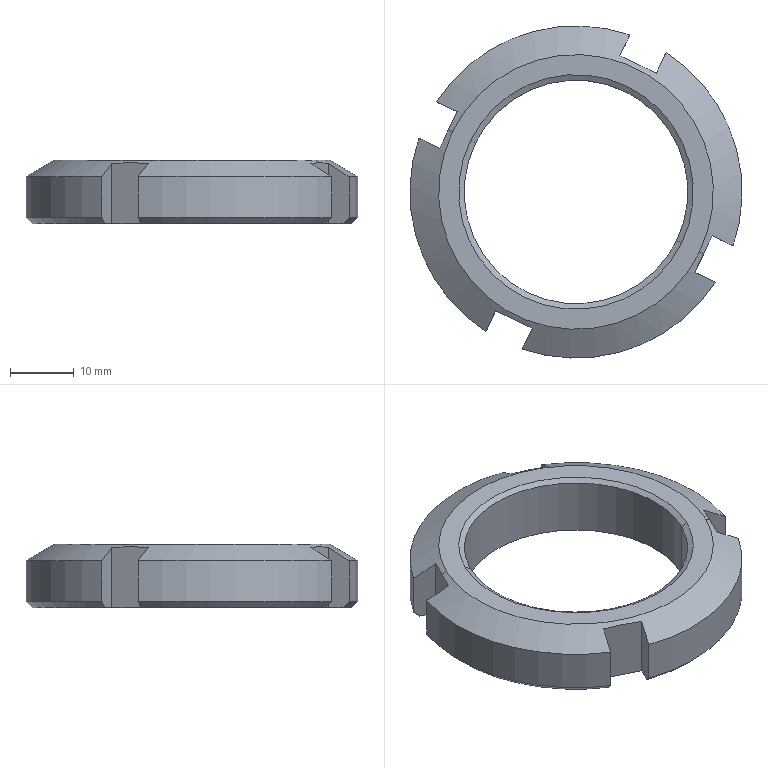Component | SolidWorks | GB812RoundNutM35_1.5-1 | 1 solid | 30 faces | box 52 x 52 x 10 mm | volume 9804 mm3 | plane 14 | cone 10 | cylinder 6 | commonest cylinder face diameters 52 x4 35 x2 | material A3
STEP:
#1=COLOUR_RGB('',0.7922,0.8196,0.9333);
#2=FILL_AREA_STYLE_COLOUR('',#1);
#3=FILL_AREA_STYLE('',(#2));
#4=SURFACE_STYLE_FILL_AREA(#3);
#5=SURFACE_SIDE_STYLE('',(#4));
#6=SURFACE_STYLE_USAGE(.BOTH.,#5);
#7=PRESENTATION_STYLE_ASSIGNMENT((#6));
#8=CARTESIAN_POINT('',(28.24,8.203,-0.07874));
#9=VERTEX_POINT('',#8);
#10=CARTESIAN_POINT('',(29.479,7.602,-0.07874));
#11=VERTEX_POINT('',#10);
#12=CARTESIAN_POINT('',(28.859,7.902,-0.07874));
#13=DIRECTION('',(0.,-0.,-1.));
#14=DIRECTION('',(0.8996,-0.4367,0.));
#15=AXIS2_PLACEMENT_3D('',#12,#13,#14);
#16=CIRCLE('',#15,0.689);
#17=EDGE_CURVE('',#9,#11,#16,.T.);
#18=ORIENTED_EDGE('',*,*,#17,.F.);
#19=CARTESIAN_POINT('',(28.209,8.218,-0.09843));
#20=VERTEX_POINT('',#19);
#21=CARTESIAN_POINT('',(28.24,8.203,-0.07874));
#22=DIRECTION('',(-0.7791,0.3782,-0.5));
#23=VECTOR('',#22,39.37);
#24=LINE('',#21,#23);
#25=EDGE_CURVE('',#9,#20,#24,.T.);
#26=ORIENTED_EDGE('',*,*,#25,.T.);
#27=CARTESIAN_POINT('',(29.51,7.587,-0.09843));
#28=VERTEX_POINT('',#27);
#29=CARTESIAN_POINT('',(28.859,7.902,-0.09843));
#30=DIRECTION('',(-0.,0.,1.));
#31=DIRECTION('',(0.8996,-0.4367,0.));
#32=AXIS2_PLACEMENT_3D('',#29,#30,#31);
#33=CIRCLE('',#32,0.7231);
#34=EDGE_CURVE('',#28,#20,#33,.T.);
#35=ORIENTED_EDGE('',*,*,#34,.F.);
#36=CARTESIAN_POINT('',(29.479,7.602,-0.07874));
#37=DIRECTION('',(0.7791,-0.3782,-0.5));
#38=VECTOR('',#37,39.37);
#39=LINE('',#36,#38);
#40=EDGE_CURVE('',#11,#28,#39,.T.);
#41=ORIENTED_EDGE('',*,*,#40,.F.);
#42=EDGE_LOOP('',(#18,#26,#35,#41));
#43=FACE_OUTER_BOUND('',#42,.T.);
#44=CARTESIAN_POINT('',(28.859,7.902,-0.07874));
#45=DIRECTION('',(0.,-0.,-1.));
#46=DIRECTION('',(0.8996,-0.4367,0.));
#47=AXIS2_PLACEMENT_3D('',#44,#45,#46);
#48=CONICAL_SURFACE('',#47,0.689,1.047);
#49=ADVANCED_FACE('',(#43),#48,.F.);
#50=CARTESIAN_POINT('',(29.479,7.602,0.2756));
#51=VERTEX_POINT('',#50);
#52=CARTESIAN_POINT('',(28.24,8.203,0.2756));
#53=VERTEX_POINT('',#52);
#54=CARTESIAN_POINT('',(28.859,7.902,0.2756));
#55=DIRECTION('',(-0.,0.,1.));
#56=DIRECTION('',(0.8996,-0.4367,0.));
#57=AXIS2_PLACEMENT_3D('',#54,#55,#56);
#58=CIRCLE('',#57,0.689);
#59=EDGE_CURVE('',#51,#53,#58,.T.);
#60=ORIENTED_EDGE('',*,*,#59,.F.);
#61=CARTESIAN_POINT('',(29.51,7.587,0.2953));
#62=VERTEX_POINT('',#61);
#63=CARTESIAN_POINT('',(29.51,7.587,0.2953));
#64=DIRECTION('',(0.7791,-0.3782,0.5));
#65=VECTOR('',#64,39.37);
#66=LINE('',#63,#65);
#67=EDGE_CURVE('',#51,#62,#66,.T.);
#68=ORIENTED_EDGE('',*,*,#67,.T.);
#69=CARTESIAN_POINT('',(28.209,8.218,0.2953));
#70=VERTEX_POINT('',#69);
#71=CARTESIAN_POINT('',(28.859,7.902,0.2953));
#72=DIRECTION('',(0.,-0.,-1.));
#73=DIRECTION('',(0.8996,-0.4367,0.));
#74=AXIS2_PLACEMENT_3D('',#71,#72,#73);
#75=CIRCLE('',#74,0.7231);
#76=EDGE_CURVE('',#70,#62,#75,.T.);
#77=ORIENTED_EDGE('',*,*,#76,.F.);
#78=CARTESIAN_POINT('',(28.209,8.218,0.2953));
#79=DIRECTION('',(-0.7791,0.3782,0.5));
#80=VECTOR('',#79,39.37);
#81=LINE('',#78,#80);
#82=EDGE_CURVE('',#53,#70,#81,.T.);
#83=ORIENTED_EDGE('',*,*,#82,.F.);
#84=EDGE_LOOP('',(#60,#68,#77,#83));
#85=FACE_OUTER_BOUND('',#84,.T.);
#86=CARTESIAN_POINT('',(28.859,7.902,0.2953));
#87=DIRECTION('',(-0.,0.,1.));
#88=DIRECTION('',(-0.8996,0.4367,-0.));
#89=AXIS2_PLACEMENT_3D('',#86,#87,#88);
#90=CONICAL_SURFACE('',#89,0.7231,1.047);
#91=ADVANCED_FACE('',(#85),#90,.F.);
#92=CARTESIAN_POINT('',(28.098,8.272,0.2953));
#93=VERTEX_POINT('',#92);
#94=CARTESIAN_POINT('',(29.621,7.533,0.2953));
#95=VERTEX_POINT('',#94);
#96=CARTESIAN_POINT('',(28.859,7.902,0.2953));
#97=DIRECTION('',(-0.,0.,1.));
#98=DIRECTION('',(0.8996,-0.4367,0.));
#99=AXIS2_PLACEMENT_3D('',#96,#97,#98);
#100=CIRCLE('',#99,0.8465);
#101=EDGE_CURVE('',#93,#95,#100,.T.);
#102=ORIENTED_EDGE('',*,*,#101,.F.);
#103=CARTESIAN_POINT('',(28.073,8.284,0.2792));
#104=VERTEX_POINT('',#103);
#105=CARTESIAN_POINT('',(27.939,8.349,0.193));
#106=DIRECTION('',(-0.7791,0.3782,-0.5));
#107=VECTOR('',#106,39.37);
#108=LINE('',#105,#107);
#109=EDGE_CURVE('',#93,#104,#108,.T.);
#110=ORIENTED_EDGE('',*,*,#109,.T.);
#111=CARTESIAN_POINT('',(28.019,8.173,0.2741));
#112=VERTEX_POINT('',#111);
#113=CARTESIAN_POINT('',(28.019,8.173,0.2741));
#114=CARTESIAN_POINT('',(28.037,8.21,0.2775));
#115=CARTESIAN_POINT('',(28.055,8.247,0.2792));
#116=CARTESIAN_POINT('',(28.073,8.284,0.2792));
#117=B_SPLINE_CURVE_WITH_KNOTS('',3,(#113,#114,#115,#116),.UNSPECIFIED.,.F.,.F.,(4,4),(0.006603,0.009752),.UNSPECIFIED.);
#118=EDGE_CURVE('',#112,#104,#117,.T.);
#119=ORIENTED_EDGE('',*,*,#118,.F.);
#120=CARTESIAN_POINT('',(27.891,8.235,0.193));
#121=VERTEX_POINT('',#120);
#122=CARTESIAN_POINT('',(27.891,8.235,0.193));
#123=CARTESIAN_POINT('',(27.934,8.214,0.2201));
#124=CARTESIAN_POINT('',(27.976,8.193,0.2471));
#125=CARTESIAN_POINT('',(28.019,8.173,0.2741));
#126=B_SPLINE_CURVE_WITH_KNOTS('',3,(#122,#123,#124,#125),.UNSPECIFIED.,.F.,.F.,(4,4),(0.007772,0.01192),.UNSPECIFIED.);
#127=EDGE_CURVE('',#121,#112,#126,.T.);
#128=ORIENTED_EDGE('',*,*,#127,.F.);
#129=CARTESIAN_POINT('',(28.304,7.043,0.193));
#130=VERTEX_POINT('',#129);
#131=CARTESIAN_POINT('',(28.859,7.902,0.193));
#132=DIRECTION('',(0.,-0.,-1.));
#133=DIRECTION('',(0.8996,-0.4367,0.));
#134=AXIS2_PLACEMENT_3D('',#131,#132,#133);
#135=CIRCLE('',#134,1.024);
#136=EDGE_CURVE('',#130,#121,#135,.T.);
#137=ORIENTED_EDGE('',*,*,#136,.F.);
#138=CARTESIAN_POINT('',(28.366,7.17,0.2741));
#139=VERTEX_POINT('',#138);
#140=CARTESIAN_POINT('',(28.366,7.17,0.2741));
#141=CARTESIAN_POINT('',(28.345,7.128,0.2471));
#142=CARTESIAN_POINT('',(28.325,7.085,0.2201));
#143=CARTESIAN_POINT('',(28.304,7.043,0.193));
#144=B_SPLINE_CURVE_WITH_KNOTS('',3,(#140,#141,#142,#143),.UNSPECIFIED.,.F.,.F.,(4,4),(0.008039,0.01219),.UNSPECIFIED.);
#145=EDGE_CURVE('',#139,#130,#144,.T.);
#146=ORIENTED_EDGE('',*,*,#145,.F.);
#147=CARTESIAN_POINT('',(28.589,7.062,0.2741));
#148=VERTEX_POINT('',#147);
#149=CARTESIAN_POINT('',(28.589,7.062,0.2741));
#150=CARTESIAN_POINT('',(28.552,7.08,0.2774));
#151=CARTESIAN_POINT('',(28.515,7.098,0.2792));
#152=CARTESIAN_POINT('',(28.459,7.125,0.2792));
#153=CARTESIAN_POINT('',(28.441,7.134,0.2788));
#154=CARTESIAN_POINT('',(28.403,7.152,0.2771));
#155=CARTESIAN_POINT('',(28.385,7.161,0.2758));
#156=CARTESIAN_POINT('',(28.366,7.17,0.2741));
#157=B_SPLINE_CURVE_WITH_KNOTS('',3,(#149,#150,#151,#152,#153,#154,#155,#156),.UNSPECIFIED.,.F.,.F.,(4,2,2,4),(0.006603,0.009741,0.01131,0.01288),.UNSPECIFIED.);
#158=EDGE_CURVE('',#148,#139,#157,.T.);
#159=ORIENTED_EDGE('',*,*,#158,.F.);
#160=CARTESIAN_POINT('',(28.527,6.934,0.193));
#161=VERTEX_POINT('',#160);
#162=CARTESIAN_POINT('',(28.527,6.934,0.193));
#163=CARTESIAN_POINT('',(28.548,6.977,0.2201));
#164=CARTESIAN_POINT('',(28.568,7.019,0.2471));
#165=CARTESIAN_POINT('',(28.589,7.062,0.2741));
#166=B_SPLINE_CURVE_WITH_KNOTS('',3,(#162,#163,#164,#165),.UNSPECIFIED.,.F.,.F.,(4,4),(0.004784,0.008932),.UNSPECIFIED.);
#167=EDGE_CURVE('',#161,#148,#166,.T.);
#168=ORIENTED_EDGE('',*,*,#167,.F.);
#169=CARTESIAN_POINT('',(29.719,7.347,0.193));
#170=VERTEX_POINT('',#169);
#171=CARTESIAN_POINT('',(28.859,7.902,0.193));
#172=DIRECTION('',(0.,-0.,-1.));
#173=DIRECTION('',(0.8996,-0.4367,0.));
#174=AXIS2_PLACEMENT_3D('',#171,#172,#173);
#175=CIRCLE('',#174,1.024);
#176=EDGE_CURVE('',#170,#161,#175,.T.);
#177=ORIENTED_EDGE('',*,*,#176,.F.);
#178=CARTESIAN_POINT('',(29.592,7.409,0.2741));
#179=VERTEX_POINT('',#178);
#180=CARTESIAN_POINT('',(29.592,7.409,0.2741));
#181=CARTESIAN_POINT('',(29.634,7.388,0.2471));
#182=CARTESIAN_POINT('',(29.677,7.368,0.2201));
#183=CARTESIAN_POINT('',(29.719,7.347,0.193));
#184=B_SPLINE_CURVE_WITH_KNOTS('',3,(#180,#181,#182,#183),.UNSPECIFIED.,.F.,.F.,(4,4),(0.008039,0.01219),.UNSPECIFIED.);
#185=EDGE_CURVE('',#179,#170,#184,.T.);
#186=ORIENTED_EDGE('',*,*,#185,.F.);
#187=CARTESIAN_POINT('',(29.646,7.521,0.2792));
#188=VERTEX_POINT('',#187);
#189=CARTESIAN_POINT('',(29.646,7.521,0.2792));
#190=CARTESIAN_POINT('',(29.628,7.483,0.2792));
#191=CARTESIAN_POINT('',(29.61,7.446,0.2775));
#192=CARTESIAN_POINT('',(29.592,7.409,0.2741));
#193=B_SPLINE_CURVE_WITH_KNOTS('',3,(#189,#190,#191,#192),.UNSPECIFIED.,.F.,.F.,(4,4),(0.01618,0.01933),.UNSPECIFIED.);
#194=EDGE_CURVE('',#188,#179,#193,.T.);
#195=ORIENTED_EDGE('',*,*,#194,.F.);
#196=CARTESIAN_POINT('',(29.78,7.455,0.193));
#197=DIRECTION('',(0.7791,-0.3782,-0.5));
#198=VECTOR('',#197,39.37);
#199=LINE('',#196,#198);
#200=EDGE_CURVE('',#95,#188,#199,.T.);
#201=ORIENTED_EDGE('',*,*,#200,.F.);
#202=EDGE_LOOP('',(#102,#110,#119,#128,#137,#146,#159,#168,#177,#186,#195,#201));
#203=FACE_OUTER_BOUND('',#202,.T.);
#204=CARTESIAN_POINT('',(28.859,7.902,0.193));
#205=DIRECTION('',(0.,-0.,-1.));
#206=DIRECTION('',(0.8996,-0.4367,0.));
#207=AXIS2_PLACEMENT_3D('',#204,#205,#206);
#208=CONICAL_SURFACE('',#207,1.024,1.047);
#209=ADVANCED_FACE('',(#203),#208,.T.);
#210=ORIENTED_EDGE('',*,*,#17,.T.);
#211=CARTESIAN_POINT('',(29.479,7.602,-0.09843));
#212=DIRECTION('',(-0.,0.,1.));
#213=VECTOR('',#212,39.37);
#214=LINE('',#211,#213);
#215=EDGE_CURVE('',#11,#51,#214,.T.);
#216=ORIENTED_EDGE('',*,*,#215,.T.);
#217=ORIENTED_EDGE('',*,*,#59,.T.);
#218=CARTESIAN_POINT('',(28.24,8.203,-0.09843));
#219=DIRECTION('',(-0.,0.,1.));
#220=VECTOR('',#219,39.37);
#221=LINE('',#218,#220);
#222=EDGE_CURVE('',#9,#53,#221,.T.);
#223=ORIENTED_EDGE('',*,*,#222,.F.);
#224=EDGE_LOOP('',(#210,#216,#217,#223));
#225=FACE_OUTER_BOUND('',#224,.T.);
#226=CARTESIAN_POINT('',(28.859,7.902,-0.09843));
#227=DIRECTION('',(-0.,0.,1.));
#228=DIRECTION('',(-0.8996,0.4367,-0.));
#229=AXIS2_PLACEMENT_3D('',#226,#227,#228);
#230=CYLINDRICAL_SURFACE('',#229,0.689);
#231=ADVANCED_FACE('',(#225),#230,.F.);
#232=CARTESIAN_POINT('',(28.527,6.934,-0.05906));
#233=VERTEX_POINT('',#232);
#234=CARTESIAN_POINT('',(29.719,7.347,-0.05906));
#235=VERTEX_POINT('',#234);
#236=CARTESIAN_POINT('',(28.859,7.902,-0.05906));
#237=DIRECTION('',(-0.,0.,1.));
#238=DIRECTION('',(0.8996,-0.4367,0.));
#239=AXIS2_PLACEMENT_3D('',#236,#237,#238);
#240=CIRCLE('',#239,1.024);
#241=EDGE_CURVE('',#233,#235,#240,.T.);
#242=ORIENTED_EDGE('',*,*,#241,.T.);
#243=CARTESIAN_POINT('',(29.719,7.347,0.2953));
#244=DIRECTION('',(0.,-0.,-1.));
#245=VECTOR('',#244,39.37);
#246=LINE('',#243,#245);
#247=EDGE_CURVE('',#170,#235,#246,.T.);
#248=ORIENTED_EDGE('',*,*,#247,.F.);
#249=ORIENTED_EDGE('',*,*,#176,.T.);
#250=CARTESIAN_POINT('',(28.527,6.934,0.2953));
#251=DIRECTION('',(0.,-0.,-1.));
#252=VECTOR('',#251,39.37);
#253=LINE('',#250,#252);
#254=EDGE_CURVE('',#161,#233,#253,.T.);
#255=ORIENTED_EDGE('',*,*,#254,.T.);
#256=EDGE_LOOP('',(#242,#248,#249,#255));
#257=FACE_OUTER_BOUND('',#256,.T.);
#258=CARTESIAN_POINT('',(28.859,7.902,-0.09843));
#259=DIRECTION('',(-0.,0.,1.));
#260=DIRECTION('',(-0.8996,0.4367,-0.));
#261=AXIS2_PLACEMENT_3D('',#258,#259,#260);
#262=CYLINDRICAL_SURFACE('',#261,1.024);
#263=ADVANCED_FACE('',(#257),#262,.T.);
#264=CARTESIAN_POINT('',(29.684,7.364,-0.09843));
#265=VERTEX_POINT('',#264);
#266=CARTESIAN_POINT('',(29.719,7.347,-0.05906));
#267=CARTESIAN_POINT('',(29.708,7.352,-0.07117));
#268=CARTESIAN_POINT('',(29.697,7.358,-0.08329));
#269=CARTESIAN_POINT('',(29.686,7.363,-0.0954));
#270=CARTESIAN_POINT('',(29.685,7.364,-0.09641));
#271=CARTESIAN_POINT('',(29.685,7.364,-0.09742));
#272=CARTESIAN_POINT('',(29.684,7.364,-0.09843));
#273=B_SPLINE_CURVE_WITH_KNOTS('',3,(#266,#267,#268,#269,#270,#271,#272),.UNSPECIFIED.,.F.,.F.,(4,3,4),(0.00583,0.007141,0.00725),.UNSPECIFIED.);
#274=EDGE_CURVE('',#235,#265,#273,.T.);
#275=ORIENTED_EDGE('',*,*,#274,.F.);
#276=ORIENTED_EDGE('',*,*,#241,.F.);
#277=CARTESIAN_POINT('',(28.545,6.97,-0.09843));
#278=VERTEX_POINT('',#277);
#279=CARTESIAN_POINT('',(28.545,6.97,-0.09843));
#280=CARTESIAN_POINT('',(28.544,6.969,-0.09742));
#281=CARTESIAN_POINT('',(28.544,6.968,-0.09641));
#282=CARTESIAN_POINT('',(28.543,6.967,-0.0954));
#283=CARTESIAN_POINT('',(28.538,6.956,-0.08329));
#284=CARTESIAN_POINT('',(28.533,6.945,-0.07117));
#285=CARTESIAN_POINT('',(28.527,6.934,-0.05906));
#286=B_SPLINE_CURVE_WITH_KNOTS('',3,(#279,#280,#281,#282,#283,#284,#285),.UNSPECIFIED.,.F.,.F.,(4,3,4),(0.007032,0.007141,0.008451),.UNSPECIFIED.);
#287=EDGE_CURVE('',#278,#233,#286,.T.);
#288=ORIENTED_EDGE('',*,*,#287,.F.);
#289=CARTESIAN_POINT('',(28.859,7.902,-0.09843));
#290=DIRECTION('',(0.,-0.,-1.));
#291=DIRECTION('',(0.8996,-0.4367,0.));
#292=AXIS2_PLACEMENT_3D('',#289,#290,#291);
#293=CIRCLE('',#292,0.9843);
#294=EDGE_CURVE('',#265,#278,#293,.T.);
#295=ORIENTED_EDGE('',*,*,#294,.F.);
#296=EDGE_LOOP('',(#275,#276,#288,#295));
#297=FACE_OUTER_BOUND('',#296,.T.);
#298=CARTESIAN_POINT('',(28.859,7.902,-0.09843));
#299=DIRECTION('',(-0.,0.,1.));
#300=DIRECTION('',(-0.8996,0.4367,-0.));
#301=AXIS2_PLACEMENT_3D('',#298,#299,#300);
#302=CONICAL_SURFACE('',#301,0.9843,0.7854);
#303=ADVANCED_FACE('',(#297),#302,.T.);
#304=CARTESIAN_POINT('',(27.891,8.235,-0.05906));
#305=VERTEX_POINT('',#304);
#306=CARTESIAN_POINT('',(28.304,7.043,-0.05906));
#307=VERTEX_POINT('',#306);
#308=CARTESIAN_POINT('',(28.859,7.902,-0.05906));
#309=DIRECTION('',(-0.,0.,1.));
#310=DIRECTION('',(0.8996,-0.4367,0.));
#311=AXIS2_PLACEMENT_3D('',#308,#309,#310);
#312=CIRCLE('',#311,1.024);
#313=EDGE_CURVE('',#305,#307,#312,.T.);
#314=ORIENTED_EDGE('',*,*,#313,.T.);
#315=CARTESIAN_POINT('',(28.304,7.043,0.2953));
#316=DIRECTION('',(0.,-0.,-1.));
#317=VECTOR('',#316,39.37);
#318=LINE('',#315,#317);
#319=EDGE_CURVE('',#130,#307,#318,.T.);
#320=ORIENTED_EDGE('',*,*,#319,.F.);
#321=ORIENTED_EDGE('',*,*,#136,.T.);
#322=CARTESIAN_POINT('',(27.891,8.235,0.2953));
#323=DIRECTION('',(0.,-0.,-1.));
#324=VECTOR('',#323,39.37);
#325=LINE('',#322,#324);
#326=EDGE_CURVE('',#121,#305,#325,.T.);
#327=ORIENTED_EDGE('',*,*,#326,.T.);
#328=EDGE_LOOP('',(#314,#320,#321,#327));
#329=FACE_OUTER_BOUND('',#328,.T.);
#330=CARTESIAN_POINT('',(28.859,7.902,-0.09843));
#331=DIRECTION('',(-0.,0.,1.));
#332=DIRECTION('',(-0.8996,0.4367,-0.));
#333=AXIS2_PLACEMENT_3D('',#330,#331,#332);
#334=CYLINDRICAL_SURFACE('',#333,1.024);
#335=ADVANCED_FACE('',(#329),#334,.T.);
#336=CARTESIAN_POINT('',(28.321,7.078,-0.09843));
#337=VERTEX_POINT('',#336);
#338=CARTESIAN_POINT('',(28.304,7.043,-0.05906));
#339=CARTESIAN_POINT('',(28.309,7.054,-0.07117));
#340=CARTESIAN_POINT('',(28.315,7.065,-0.08329));
#341=CARTESIAN_POINT('',(28.32,7.075,-0.0954));
#342=CARTESIAN_POINT('',(28.321,7.076,-0.09641));
#343=CARTESIAN_POINT('',(28.321,7.077,-0.09742));
#344=CARTESIAN_POINT('',(28.321,7.078,-0.09843));
#345=B_SPLINE_CURVE_WITH_KNOTS('',3,(#338,#339,#340,#341,#342,#343,#344),.UNSPECIFIED.,.F.,.F.,(4,3,4),(0.00583,0.007141,0.00725),.UNSPECIFIED.);
#346=EDGE_CURVE('',#307,#337,#345,.T.);
#347=ORIENTED_EDGE('',*,*,#346,.F.);
#348=ORIENTED_EDGE('',*,*,#313,.F.);
#349=CARTESIAN_POINT('',(27.927,8.217,-0.09843));
#350=VERTEX_POINT('',#349);
#351=CARTESIAN_POINT('',(27.927,8.217,-0.09843));
#352=CARTESIAN_POINT('',(27.921,8.22,-0.09151));
#353=CARTESIAN_POINT('',(27.914,8.223,-0.0846));
#354=CARTESIAN_POINT('',(27.908,8.226,-0.07768));
#355=CARTESIAN_POINT('',(27.902,8.229,-0.07147));
#356=CARTESIAN_POINT('',(27.897,8.232,-0.06526));
#357=CARTESIAN_POINT('',(27.891,8.235,-0.05906));
#358=B_SPLINE_CURVE_WITH_KNOTS('',3,(#351,#352,#353,#354,#355,#356,#357),.UNSPECIFIED.,.F.,.F.,(4,3,4),(0.006393,0.007141,0.007812),.UNSPECIFIED.);
#359=EDGE_CURVE('',#350,#305,#358,.T.);
#360=ORIENTED_EDGE('',*,*,#359,.F.);
#361=CARTESIAN_POINT('',(28.859,7.902,-0.09843));
#362=DIRECTION('',(0.,-0.,-1.));
#363=DIRECTION('',(0.8996,-0.4367,0.));
#364=AXIS2_PLACEMENT_3D('',#361,#362,#363);
#365=CIRCLE('',#364,0.9843);
#366=EDGE_CURVE('',#337,#350,#365,.T.);
#367=ORIENTED_EDGE('',*,*,#366,.F.);
#368=EDGE_LOOP('',(#347,#348,#360,#367));
#369=FACE_OUTER_BOUND('',#368,.T.);
#370=CARTESIAN_POINT('',(28.859,7.902,-0.09843));
#371=DIRECTION('',(-0.,0.,1.));
#372=DIRECTION('',(-0.8996,0.4367,-0.));
#373=AXIS2_PLACEMENT_3D('',#370,#371,#372);
#374=CONICAL_SURFACE('',#373,0.9843,0.7854);
#375=ADVANCED_FACE('',(#369),#374,.T.);
#376=CARTESIAN_POINT('',(29.192,8.871,-0.05906));
#377=VERTEX_POINT('',#376);
#378=CARTESIAN_POINT('',(28.,8.458,-0.05906));
#379=VERTEX_POINT('',#378);
#380=CARTESIAN_POINT('',(28.859,7.902,-0.05906));
#381=DIRECTION('',(-0.,0.,1.));
#382=DIRECTION('',(0.8996,-0.4367,0.));
#383=AXIS2_PLACEMENT_3D('',#380,#381,#382);
#384=CIRCLE('',#383,1.024);
#385=EDGE_CURVE('',#377,#379,#384,.T.);
#386=ORIENTED_EDGE('',*,*,#385,.T.);
#387=CARTESIAN_POINT('',(28.,8.458,0.193));
#388=VERTEX_POINT('',#387);
#389=CARTESIAN_POINT('',(28.,8.458,0.2953));
#390=DIRECTION('',(0.,-0.,-1.));
#391=VECTOR('',#390,39.37);
#392=LINE('',#389,#391);
#393=EDGE_CURVE('',#388,#379,#392,.T.);
#394=ORIENTED_EDGE('',*,*,#393,.F.);
#395=CARTESIAN_POINT('',(29.192,8.871,0.193));
#396=VERTEX_POINT('',#395);
#397=CARTESIAN_POINT('',(28.859,7.902,0.193));
#398=DIRECTION('',(0.,-0.,-1.));
#399=DIRECTION('',(0.8996,-0.4367,0.));
#400=AXIS2_PLACEMENT_3D('',#397,#398,#399);
#401=CIRCLE('',#400,1.024);
#402=EDGE_CURVE('',#388,#396,#401,.T.);
#403=ORIENTED_EDGE('',*,*,#402,.T.);
#404=CARTESIAN_POINT('',(29.192,8.871,0.2953));
#405=DIRECTION('',(0.,-0.,-1.));
#406=VECTOR('',#405,39.37);
#407=LINE('',#404,#406);
#408=EDGE_CURVE('',#396,#377,#407,.T.);
#409=ORIENTED_EDGE('',*,*,#408,.T.);
#410=EDGE_LOOP('',(#386,#394,#403,#409));
#411=FACE_OUTER_BOUND('',#410,.T.);
#412=CARTESIAN_POINT('',(28.859,7.902,-0.09843));
#413=DIRECTION('',(-0.,0.,1.));
#414=DIRECTION('',(-0.8996,0.4367,-0.));
#415=AXIS2_PLACEMENT_3D('',#412,#413,#414);
#416=CYLINDRICAL_SURFACE('',#415,1.024);
#417=ADVANCED_FACE('',(#411),#416,.T.);
#418=CARTESIAN_POINT('',(28.035,8.44,-0.09843));
#419=VERTEX_POINT('',#418);
#420=CARTESIAN_POINT('',(28.,8.458,-0.05906));
#421=CARTESIAN_POINT('',(28.005,8.455,-0.06526));
#422=CARTESIAN_POINT('',(28.011,8.452,-0.07147));
#423=CARTESIAN_POINT('',(28.016,8.45,-0.07768));
#424=CARTESIAN_POINT('',(28.023,8.447,-0.0846));
#425=CARTESIAN_POINT('',(28.029,8.443,-0.09151));
#426=CARTESIAN_POINT('',(28.035,8.44,-0.09843));
#427=B_SPLINE_CURVE_WITH_KNOTS('',3,(#420,#421,#422,#423,#424,#425,#426),.UNSPECIFIED.,.F.,.F.,(4,3,4),(0.006469,0.007141,0.007889),.UNSPECIFIED.);
#428=EDGE_CURVE('',#379,#419,#427,.T.);
#429=ORIENTED_EDGE('',*,*,#428,.F.);
#430=ORIENTED_EDGE('',*,*,#385,.F.);
#431=CARTESIAN_POINT('',(29.174,8.835,-0.09843));
#432=VERTEX_POINT('',#431);
#433=CARTESIAN_POINT('',(29.174,8.835,-0.09843));
#434=CARTESIAN_POINT('',(29.177,8.841,-0.09151));
#435=CARTESIAN_POINT('',(29.18,8.847,-0.0846));
#436=CARTESIAN_POINT('',(29.183,8.854,-0.07768));
#437=CARTESIAN_POINT('',(29.186,8.859,-0.07147));
#438=CARTESIAN_POINT('',(29.189,8.865,-0.06526));
#439=CARTESIAN_POINT('',(29.192,8.871,-0.05906));
#440=B_SPLINE_CURVE_WITH_KNOTS('',3,(#433,#434,#435,#436,#437,#438,#439),.UNSPECIFIED.,.F.,.F.,(4,3,4),(0.006393,0.007141,0.007812),.UNSPECIFIED.);
#441=EDGE_CURVE('',#432,#377,#440,.T.);
#442=ORIENTED_EDGE('',*,*,#441,.F.);
#443=CARTESIAN_POINT('',(28.859,7.902,-0.09843));
#444=DIRECTION('',(0.,-0.,-1.));
#445=DIRECTION('',(0.8996,-0.4367,0.));
#446=AXIS2_PLACEMENT_3D('',#443,#444,#445);
#447=CIRCLE('',#446,0.9843);
#448=EDGE_CURVE('',#419,#432,#447,.T.);
#449=ORIENTED_EDGE('',*,*,#448,.F.);
#450=EDGE_LOOP('',(#429,#430,#442,#449));
#451=FACE_OUTER_BOUND('',#450,.T.);
#452=CARTESIAN_POINT('',(28.859,7.902,-0.09843));
#453=DIRECTION('',(-0.,0.,1.));
#454=DIRECTION('',(-0.8996,0.4367,-0.));
#455=AXIS2_PLACEMENT_3D('',#452,#453,#454);
#456=CONICAL_SURFACE('',#455,0.9843,0.7854);
#457=ADVANCED_FACE('',(#451),#456,.T.);
#458=ORIENTED_EDGE('',*,*,#34,.T.);
#459=CARTESIAN_POINT('',(28.859,7.902,-0.09843));
#460=DIRECTION('',(-0.,0.,1.));
#461=DIRECTION('',(0.8996,-0.4367,0.));
#462=AXIS2_PLACEMENT_3D('',#459,#460,#461);
#463=CIRCLE('',#462,0.7231);
#464=EDGE_CURVE('',#20,#28,#463,.T.);
#465=ORIENTED_EDGE('',*,*,#464,.T.);
#466=EDGE_LOOP('',(#458,#465));
#467=FACE_BOUND('',#466,.T.);
#468=CARTESIAN_POINT('',(29.592,7.409,-0.09843));
#469=VERTEX_POINT('',#468);
#470=CARTESIAN_POINT('',(29.592,7.409,-0.09843));
#471=DIRECTION('',(-0.8996,0.4367,-0.));
#472=VECTOR('',#471,39.37);
#473=LINE('',#470,#472);
#474=EDGE_CURVE('',#265,#469,#473,.T.);
#475=ORIENTED_EDGE('',*,*,#474,.F.);
#476=ORIENTED_EDGE('',*,*,#294,.T.);
#477=CARTESIAN_POINT('',(28.589,7.062,-0.09843));
#478=VERTEX_POINT('',#477);
#479=CARTESIAN_POINT('',(28.589,7.062,-0.09843));
#480=DIRECTION('',(-0.4367,-0.8996,0.));
#481=VECTOR('',#480,39.37);
#482=LINE('',#479,#481);
#483=EDGE_CURVE('',#478,#278,#482,.T.);
#484=ORIENTED_EDGE('',*,*,#483,.F.);
#485=CARTESIAN_POINT('',(28.366,7.17,-0.09843));
#486=VERTEX_POINT('',#485);
#487=CARTESIAN_POINT('',(28.589,7.062,-0.09843));
#488=DIRECTION('',(0.8996,-0.4367,0.));
#489=VECTOR('',#488,39.37);
#490=LINE('',#487,#489);
#491=EDGE_CURVE('',#486,#478,#490,.T.);
#492=ORIENTED_EDGE('',*,*,#491,.F.);
#493=CARTESIAN_POINT('',(28.366,7.17,-0.09843));
#494=DIRECTION('',(0.4367,0.8996,-0.));
#495=VECTOR('',#494,39.37);
#496=LINE('',#493,#495);
#497=EDGE_CURVE('',#337,#486,#496,.T.);
#498=ORIENTED_EDGE('',*,*,#497,.F.);
#499=ORIENTED_EDGE('',*,*,#366,.T.);
#500=CARTESIAN_POINT('',(28.019,8.173,-0.09843));
#501=VERTEX_POINT('',#500);
#502=CARTESIAN_POINT('',(28.019,8.173,-0.09843));
#503=DIRECTION('',(-0.8996,0.4367,-0.));
#504=VECTOR('',#503,39.37);
#505=LINE('',#502,#504);
#506=EDGE_CURVE('',#501,#350,#505,.T.);
#507=ORIENTED_EDGE('',*,*,#506,.F.);
#508=CARTESIAN_POINT('',(28.127,8.396,-0.09843));
#509=VERTEX_POINT('',#508);
#510=CARTESIAN_POINT('',(28.019,8.173,-0.09843));
#511=DIRECTION('',(-0.4367,-0.8996,0.));
#512=VECTOR('',#511,39.37);
#513=LINE('',#510,#512);
#514=EDGE_CURVE('',#509,#501,#513,.T.);
#515=ORIENTED_EDGE('',*,*,#514,.F.);
#516=CARTESIAN_POINT('',(28.127,8.396,-0.09843));
#517=DIRECTION('',(0.8996,-0.4367,0.));
#518=VECTOR('',#517,39.37);
#519=LINE('',#516,#518);
#520=EDGE_CURVE('',#419,#509,#519,.T.);
#521=ORIENTED_EDGE('',*,*,#520,.F.);
#522=ORIENTED_EDGE('',*,*,#448,.T.);
#523=CARTESIAN_POINT('',(29.13,8.743,-0.09843));
#524=VERTEX_POINT('',#523);
#525=CARTESIAN_POINT('',(29.13,8.743,-0.09843));
#526=DIRECTION('',(0.4367,0.8996,-0.));
#527=VECTOR('',#526,39.37);
#528=LINE('',#525,#527);
#529=EDGE_CURVE('',#524,#432,#528,.T.);
#530=ORIENTED_EDGE('',*,*,#529,.F.);
#531=CARTESIAN_POINT('',(29.353,8.635,-0.09843));
#532=VERTEX_POINT('',#531);
#533=CARTESIAN_POINT('',(29.13,8.743,-0.09843));
#534=DIRECTION('',(-0.8996,0.4367,-0.));
#535=VECTOR('',#534,39.37);
#536=LINE('',#533,#535);
#537=EDGE_CURVE('',#532,#524,#536,.T.);
#538=ORIENTED_EDGE('',*,*,#537,.F.);
#539=CARTESIAN_POINT('',(29.397,8.727,-0.09843));
#540=VERTEX_POINT('',#539);
#541=CARTESIAN_POINT('',(29.353,8.635,-0.09843));
#542=DIRECTION('',(-0.4367,-0.8996,0.));
#543=VECTOR('',#542,39.37);
#544=LINE('',#541,#543);
#545=EDGE_CURVE('',#540,#532,#544,.T.);
#546=ORIENTED_EDGE('',*,*,#545,.F.);
#547=CARTESIAN_POINT('',(29.792,7.588,-0.09843));
#548=VERTEX_POINT('',#547);
#549=CARTESIAN_POINT('',(28.859,7.902,-0.09843));
#550=DIRECTION('',(0.,-0.,-1.));
#551=DIRECTION('',(0.8996,-0.4367,0.));
#552=AXIS2_PLACEMENT_3D('',#549,#550,#551);
#553=CIRCLE('',#552,0.9843);
#554=EDGE_CURVE('',#540,#548,#553,.T.);
#555=ORIENTED_EDGE('',*,*,#554,.T.);
#556=CARTESIAN_POINT('',(29.7,7.632,-0.09843));
#557=VERTEX_POINT('',#556);
#558=CARTESIAN_POINT('',(29.7,7.632,-0.09843));
#559=DIRECTION('',(0.8996,-0.4367,0.));
#560=VECTOR('',#559,39.37);
#561=LINE('',#558,#560);
#562=EDGE_CURVE('',#557,#548,#561,.T.);
#563=ORIENTED_EDGE('',*,*,#562,.F.);
#564=CARTESIAN_POINT('',(29.7,7.632,-0.09843));
#565=DIRECTION('',(0.4367,0.8996,-0.));
#566=VECTOR('',#565,39.37);
#567=LINE('',#564,#566);
#568=EDGE_CURVE('',#469,#557,#567,.T.);
#569=ORIENTED_EDGE('',*,*,#568,.F.);
#570=EDGE_LOOP('',(#475,#476,#484,#492,#498,#499,#507,#515,#521,#522,#530,#538,#546,#555,#563,#569));
#571=FACE_OUTER_BOUND('',#570,.T.);
#572=CARTESIAN_POINT('',(28.859,7.902,-0.09843));
#573=DIRECTION('',(0.,-0.,-1.));
#574=DIRECTION('',(0.8996,-0.4367,0.));
#575=AXIS2_PLACEMENT_3D('',#572,#573,#574);
#576=PLANE('',#575);
#577=ADVANCED_FACE('',(#467,#571),#576,.T.);
#578=ORIENTED_EDGE('',*,*,#76,.T.);
#579=CARTESIAN_POINT('',(28.859,7.902,0.2953));
#580=DIRECTION('',(0.,-0.,-1.));
#581=DIRECTION('',(0.8996,-0.4367,0.));
#582=AXIS2_PLACEMENT_3D('',#579,#580,#581);
#583=CIRCLE('',#582,0.7231);
#584=EDGE_CURVE('',#62,#70,#583,.T.);
#585=ORIENTED_EDGE('',*,*,#584,.T.);
#586=EDGE_LOOP('',(#578,#585));
#587=FACE_BOUND('',#586,.T.);
#588=CARTESIAN_POINT('',(28.859,7.902,0.2953));
#589=DIRECTION('',(-0.,0.,1.));
#590=DIRECTION('',(0.8996,-0.4367,0.));
#591=AXIS2_PLACEMENT_3D('',#588,#589,#590);
#592=CIRCLE('',#591,0.8465);
#593=EDGE_CURVE('',#95,#93,#592,.T.);
#594=ORIENTED_EDGE('',*,*,#593,.T.);
#595=ORIENTED_EDGE('',*,*,#101,.T.);
#596=EDGE_LOOP('',(#594,#595));
#597=FACE_OUTER_BOUND('',#596,.T.);
#598=CARTESIAN_POINT('',(28.859,7.902,0.2953));
#599=DIRECTION('',(0.,-0.,-1.));
#600=DIRECTION('',(0.8996,-0.4367,0.));
#601=AXIS2_PLACEMENT_3D('',#598,#599,#600);
#602=PLANE('',#601);
#603=ADVANCED_FACE('',(#587,#597),#602,.F.);
#604=CARTESIAN_POINT('',(29.415,8.762,0.193));
#605=VERTEX_POINT('',#604);
#606=CARTESIAN_POINT('',(29.828,7.57,0.193));
#607=VERTEX_POINT('',#606);
#608=CARTESIAN_POINT('',(28.859,7.902,0.193));
#609=DIRECTION('',(0.,-0.,-1.));
#610=DIRECTION('',(0.8996,-0.4367,0.));
#611=AXIS2_PLACEMENT_3D('',#608,#609,#610);
#612=CIRCLE('',#611,1.024);
#613=EDGE_CURVE('',#605,#607,#612,.T.);
#614=ORIENTED_EDGE('',*,*,#613,.T.);
#615=CARTESIAN_POINT('',(29.828,7.57,-0.05906));
#616=VERTEX_POINT('',#615);
#617=CARTESIAN_POINT('',(29.828,7.57,0.2953));
#618=DIRECTION('',(0.,-0.,-1.));
#619=VECTOR('',#618,39.37);
#620=LINE('',#617,#619);
#621=EDGE_CURVE('',#607,#616,#620,.T.);
#622=ORIENTED_EDGE('',*,*,#621,.T.);
#623=CARTESIAN_POINT('',(29.415,8.762,-0.05906));
#624=VERTEX_POINT('',#623);
#625=CARTESIAN_POINT('',(28.859,7.902,-0.05906));
#626=DIRECTION('',(-0.,0.,1.));
#627=DIRECTION('',(0.8996,-0.4367,0.));
#628=AXIS2_PLACEMENT_3D('',#625,#626,#627);
#629=CIRCLE('',#628,1.024);
#630=EDGE_CURVE('',#616,#624,#629,.T.);
#631=ORIENTED_EDGE('',*,*,#630,.T.);
#632=CARTESIAN_POINT('',(29.415,8.762,0.2953));
#633=DIRECTION('',(0.,-0.,-1.));
#634=VECTOR('',#633,39.37);
#635=LINE('',#632,#634);
#636=EDGE_CURVE('',#605,#624,#635,.T.);
#637=ORIENTED_EDGE('',*,*,#636,.F.);
#638=EDGE_LOOP('',(#614,#622,#631,#637));
#639=FACE_OUTER_BOUND('',#638,.T.);
#640=CARTESIAN_POINT('',(28.859,7.902,-0.09843));
#641=DIRECTION('',(-0.,0.,1.));
#642=DIRECTION('',(-0.8996,0.4367,-0.));
#643=AXIS2_PLACEMENT_3D('',#640,#641,#642);
#644=CYLINDRICAL_SURFACE('',#643,1.024);
#645=ADVANCED_FACE('',(#639),#644,.T.);
#646=ORIENTED_EDGE('',*,*,#215,.F.);
#647=CARTESIAN_POINT('',(28.859,7.902,-0.07874));
#648=DIRECTION('',(0.,-0.,-1.));
#649=DIRECTION('',(0.8996,-0.4367,0.));
#650=AXIS2_PLACEMENT_3D('',#647,#648,#649);
#651=CIRCLE('',#650,0.689);
#652=EDGE_CURVE('',#11,#9,#651,.T.);
#653=ORIENTED_EDGE('',*,*,#652,.T.);
#654=ORIENTED_EDGE('',*,*,#222,.T.);
#655=CARTESIAN_POINT('',(28.859,7.902,0.2756));
#656=DIRECTION('',(-0.,0.,1.));
#657=DIRECTION('',(0.8996,-0.4367,0.));
#658=AXIS2_PLACEMENT_3D('',#655,#656,#657);
#659=CIRCLE('',#658,0.689);
#660=EDGE_CURVE('',#53,#51,#659,.T.);
#661=ORIENTED_EDGE('',*,*,#660,.T.);
#662=EDGE_LOOP('',(#646,#653,#654,#661));
#663=FACE_OUTER_BOUND('',#662,.T.);
#664=CARTESIAN_POINT('',(28.859,7.902,-0.09843));
#665=DIRECTION('',(-0.,0.,1.));
#666=DIRECTION('',(-0.8996,0.4367,-0.));
#667=AXIS2_PLACEMENT_3D('',#664,#665,#666);
#668=CYLINDRICAL_SURFACE('',#667,0.689);
#669=ADVANCED_FACE('',(#663),#668,.F.);
#670=CARTESIAN_POINT('',(29.792,7.588,-0.09843));
#671=CARTESIAN_POINT('',(29.793,7.587,-0.09742));
#672=CARTESIAN_POINT('',(29.794,7.587,-0.09641));
#673=CARTESIAN_POINT('',(29.795,7.586,-0.0954));
#674=CARTESIAN_POINT('',(29.806,7.581,-0.08329));
#675=CARTESIAN_POINT('',(29.817,7.576,-0.07117));
#676=CARTESIAN_POINT('',(29.828,7.57,-0.05906));
#677=B_SPLINE_CURVE_WITH_KNOTS('',3,(#670,#671,#672,#673,#674,#675,#676),.UNSPECIFIED.,.F.,.F.,(4,3,4),(0.007032,0.007141,0.008451),.UNSPECIFIED.);
#678=EDGE_CURVE('',#548,#616,#677,.T.);
#679=ORIENTED_EDGE('',*,*,#678,.F.);
#680=ORIENTED_EDGE('',*,*,#554,.F.);
#681=CARTESIAN_POINT('',(29.415,8.762,-0.05906));
#682=CARTESIAN_POINT('',(29.412,8.757,-0.06526));
#683=CARTESIAN_POINT('',(29.409,8.751,-0.07147));
#684=CARTESIAN_POINT('',(29.407,8.745,-0.07768));
#685=CARTESIAN_POINT('',(29.403,8.739,-0.0846));
#686=CARTESIAN_POINT('',(29.4,8.733,-0.09151));
#687=CARTESIAN_POINT('',(29.397,8.727,-0.09843));
#688=B_SPLINE_CURVE_WITH_KNOTS('',3,(#681,#682,#683,#684,#685,#686,#687),.UNSPECIFIED.,.F.,.F.,(4,3,4),(0.006469,0.007141,0.007889),.UNSPECIFIED.);
#689=EDGE_CURVE('',#624,#540,#688,.T.);
#690=ORIENTED_EDGE('',*,*,#689,.F.);
#691=ORIENTED_EDGE('',*,*,#630,.F.);
#692=EDGE_LOOP('',(#679,#680,#690,#691));
#693=FACE_OUTER_BOUND('',#692,.T.);
#694=CARTESIAN_POINT('',(28.859,7.902,-0.09843));
#695=DIRECTION('',(-0.,0.,1.));
#696=DIRECTION('',(-0.8996,0.4367,-0.));
#697=AXIS2_PLACEMENT_3D('',#694,#695,#696);
#698=CONICAL_SURFACE('',#697,0.9843,0.7854);
#699=ADVANCED_FACE('',(#693),#698,.T.);
#700=ORIENTED_EDGE('',*,*,#109,.F.);
#701=ORIENTED_EDGE('',*,*,#593,.F.);
#702=ORIENTED_EDGE('',*,*,#200,.T.);
#703=CARTESIAN_POINT('',(29.7,7.632,0.2741));
#704=VERTEX_POINT('',#703);
#705=CARTESIAN_POINT('',(29.7,7.632,0.2741));
#706=CARTESIAN_POINT('',(29.691,7.614,0.2758));
#707=CARTESIAN_POINT('',(29.682,7.595,0.2771));
#708=CARTESIAN_POINT('',(29.664,7.558,0.2788));
#709=CARTESIAN_POINT('',(29.655,7.539,0.2792));
#710=CARTESIAN_POINT('',(29.646,7.521,0.2792));
#711=B_SPLINE_CURVE_WITH_KNOTS('',3,(#705,#706,#707,#708,#709,#710),.UNSPECIFIED.,.F.,.F.,(4,2,4),(0.01305,0.01462,0.01618),.UNSPECIFIED.);
#712=EDGE_CURVE('',#704,#188,#711,.T.);
#713=ORIENTED_EDGE('',*,*,#712,.F.);
#714=CARTESIAN_POINT('',(29.828,7.57,0.193));
#715=CARTESIAN_POINT('',(29.785,7.591,0.2201));
#716=CARTESIAN_POINT('',(29.743,7.611,0.2471));
#717=CARTESIAN_POINT('',(29.7,7.632,0.2741));
#718=B_SPLINE_CURVE_WITH_KNOTS('',3,(#714,#715,#716,#717),.UNSPECIFIED.,.F.,.F.,(4,4),(0.004784,0.008932),.UNSPECIFIED.);
#719=EDGE_CURVE('',#607,#704,#718,.T.);
#720=ORIENTED_EDGE('',*,*,#719,.F.);
#721=ORIENTED_EDGE('',*,*,#613,.F.);
#722=CARTESIAN_POINT('',(29.353,8.635,0.2741));
#723=VERTEX_POINT('',#722);
#724=CARTESIAN_POINT('',(29.353,8.635,0.2741));
#725=CARTESIAN_POINT('',(29.373,8.677,0.2471));
#726=CARTESIAN_POINT('',(29.394,8.72,0.2201));
#727=CARTESIAN_POINT('',(29.415,8.762,0.193));
#728=B_SPLINE_CURVE_WITH_KNOTS('',3,(#724,#725,#726,#727),.UNSPECIFIED.,.F.,.F.,(4,4),(0.005051,0.009199),.UNSPECIFIED.);
#729=EDGE_CURVE('',#723,#605,#728,.T.);
#730=ORIENTED_EDGE('',*,*,#729,.F.);
#731=CARTESIAN_POINT('',(29.13,8.743,0.2741));
#732=VERTEX_POINT('',#731);
#733=CARTESIAN_POINT('',(29.13,8.743,0.2741));
#734=CARTESIAN_POINT('',(29.148,8.734,0.2758));
#735=CARTESIAN_POINT('',(29.167,8.725,0.2771));
#736=CARTESIAN_POINT('',(29.204,8.707,0.2788));
#737=CARTESIAN_POINT('',(29.223,8.698,0.2792));
#738=CARTESIAN_POINT('',(29.279,8.671,0.2792));
#739=CARTESIAN_POINT('',(29.316,8.653,0.2774));
#740=CARTESIAN_POINT('',(29.353,8.635,0.2741));
#741=B_SPLINE_CURVE_WITH_KNOTS('',3,(#733,#734,#735,#736,#737,#738,#739,#740),.UNSPECIFIED.,.F.,.F.,(4,2,2,4),(0.01305,0.01462,0.01619,0.01933),.UNSPECIFIED.);
#742=EDGE_CURVE('',#732,#723,#741,.T.);
#743=ORIENTED_EDGE('',*,*,#742,.F.);
#744=CARTESIAN_POINT('',(29.192,8.871,0.193));
#745=CARTESIAN_POINT('',(29.171,8.828,0.2201));
#746=CARTESIAN_POINT('',(29.15,8.786,0.2471));
#747=CARTESIAN_POINT('',(29.13,8.743,0.2741));
#748=B_SPLINE_CURVE_WITH_KNOTS('',3,(#744,#745,#746,#747),.UNSPECIFIED.,.F.,.F.,(4,4),(0.007772,0.01192),.UNSPECIFIED.);
#749=EDGE_CURVE('',#396,#732,#748,.T.);
#750=ORIENTED_EDGE('',*,*,#749,.F.);
#751=ORIENTED_EDGE('',*,*,#402,.F.);
#752=CARTESIAN_POINT('',(28.127,8.396,0.2741));
#753=VERTEX_POINT('',#752);
#754=CARTESIAN_POINT('',(28.127,8.396,0.2741));
#755=CARTESIAN_POINT('',(28.084,8.417,0.2471));
#756=CARTESIAN_POINT('',(28.042,8.437,0.2201));
#757=CARTESIAN_POINT('',(28.,8.458,0.193));
#758=B_SPLINE_CURVE_WITH_KNOTS('',3,(#754,#755,#756,#757),.UNSPECIFIED.,.F.,.F.,(4,4),(0.005051,0.009199),.UNSPECIFIED.);
#759=EDGE_CURVE('',#753,#388,#758,.T.);
#760=ORIENTED_EDGE('',*,*,#759,.F.);
#761=CARTESIAN_POINT('',(28.073,8.284,0.2792));
#762=CARTESIAN_POINT('',(28.082,8.303,0.2792));
#763=CARTESIAN_POINT('',(28.091,8.321,0.2788));
#764=CARTESIAN_POINT('',(28.109,8.359,0.2771));
#765=CARTESIAN_POINT('',(28.118,8.377,0.2758));
#766=CARTESIAN_POINT('',(28.127,8.396,0.2741));
#767=B_SPLINE_CURVE_WITH_KNOTS('',3,(#761,#762,#763,#764,#765,#766),.UNSPECIFIED.,.F.,.F.,(4,2,4),(0.009752,0.01132,0.01288),.UNSPECIFIED.);
#768=EDGE_CURVE('',#104,#753,#767,.T.);
#769=ORIENTED_EDGE('',*,*,#768,.F.);
#770=EDGE_LOOP('',(#700,#701,#702,#713,#720,#721,#730,#743,#750,#751,#760,#769));
#771=FACE_OUTER_BOUND('',#770,.T.);
#772=CARTESIAN_POINT('',(28.859,7.902,0.193));
#773=DIRECTION('',(0.,-0.,-1.));
#774=DIRECTION('',(0.8996,-0.4367,0.));
#775=AXIS2_PLACEMENT_3D('',#772,#773,#774);
#776=CONICAL_SURFACE('',#775,1.024,1.047);
#777=ADVANCED_FACE('',(#771),#776,.T.);
#778=ORIENTED_EDGE('',*,*,#742,.T.);
#779=CARTESIAN_POINT('',(29.353,8.635,0.2953));
#780=DIRECTION('',(0.,-0.,-1.));
#781=VECTOR('',#780,39.37);
#782=LINE('',#779,#781);
#783=EDGE_CURVE('',#723,#532,#782,.T.);
#784=ORIENTED_EDGE('',*,*,#783,.T.);
#785=ORIENTED_EDGE('',*,*,#537,.T.);
#786=CARTESIAN_POINT('',(29.13,8.743,0.2953));
#787=DIRECTION('',(0.,-0.,-1.));
#788=VECTOR('',#787,39.37);
#789=LINE('',#786,#788);
#790=EDGE_CURVE('',#732,#524,#789,.T.);
#791=ORIENTED_EDGE('',*,*,#790,.F.);
#792=EDGE_LOOP('',(#778,#784,#785,#791));
#793=FACE_OUTER_BOUND('',#792,.T.);
#794=CARTESIAN_POINT('',(29.13,8.743,0.2953));
#795=DIRECTION('',(-0.4367,-0.8996,0.));
#796=DIRECTION('',(0.,-0.,-1.));
#797=AXIS2_PLACEMENT_3D('',#794,#795,#796);
#798=PLANE('',#797);
#799=ADVANCED_FACE('',(#793),#798,.F.);
#800=ORIENTED_EDGE('',*,*,#689,.T.);
#801=ORIENTED_EDGE('',*,*,#545,.T.);
#802=ORIENTED_EDGE('',*,*,#783,.F.);
#803=ORIENTED_EDGE('',*,*,#729,.T.);
#804=ORIENTED_EDGE('',*,*,#636,.T.);
#805=EDGE_LOOP('',(#800,#801,#802,#803,#804));
#806=FACE_OUTER_BOUND('',#805,.T.);
#807=CARTESIAN_POINT('',(29.353,8.635,0.2953));
#808=DIRECTION('',(0.8996,-0.4367,0.));
#809=DIRECTION('',(-0.,0.,1.));
#810=AXIS2_PLACEMENT_3D('',#807,#808,#809);
#811=PLANE('',#810);
#812=ADVANCED_FACE('',(#806),#811,.F.);
#813=ORIENTED_EDGE('',*,*,#441,.T.);
#814=ORIENTED_EDGE('',*,*,#408,.F.);
#815=ORIENTED_EDGE('',*,*,#749,.T.);
#816=ORIENTED_EDGE('',*,*,#790,.T.);
#817=ORIENTED_EDGE('',*,*,#529,.T.);
#818=EDGE_LOOP('',(#813,#814,#815,#816,#817));
#819=FACE_OUTER_BOUND('',#818,.T.);
#820=CARTESIAN_POINT('',(29.13,8.743,0.2953));
#821=DIRECTION('',(-0.8996,0.4367,-0.));
#822=DIRECTION('',(0.,-0.,-1.));
#823=AXIS2_PLACEMENT_3D('',#820,#821,#822);
#824=PLANE('',#823);
#825=ADVANCED_FACE('',(#819),#824,.F.);
#826=ORIENTED_EDGE('',*,*,#118,.T.);
#827=ORIENTED_EDGE('',*,*,#768,.T.);
#828=CARTESIAN_POINT('',(28.127,8.396,0.2953));
#829=DIRECTION('',(0.,-0.,-1.));
#830=VECTOR('',#829,39.37);
#831=LINE('',#828,#830);
#832=EDGE_CURVE('',#753,#509,#831,.T.);
#833=ORIENTED_EDGE('',*,*,#832,.T.);
#834=ORIENTED_EDGE('',*,*,#514,.T.);
#835=CARTESIAN_POINT('',(28.019,8.173,0.2953));
#836=DIRECTION('',(0.,-0.,-1.));
#837=VECTOR('',#836,39.37);
#838=LINE('',#835,#837);
#839=EDGE_CURVE('',#112,#501,#838,.T.);
#840=ORIENTED_EDGE('',*,*,#839,.F.);
#841=EDGE_LOOP('',(#826,#827,#833,#834,#840));
#842=FACE_OUTER_BOUND('',#841,.T.);
#843=CARTESIAN_POINT('',(28.019,8.173,0.2953));
#844=DIRECTION('',(0.8996,-0.4367,0.));
#845=DIRECTION('',(-0.4367,-0.8996,0.));
#846=AXIS2_PLACEMENT_3D('',#843,#844,#845);
#847=PLANE('',#846);
#848=ADVANCED_FACE('',(#842),#847,.F.);
#849=ORIENTED_EDGE('',*,*,#428,.T.);
#850=ORIENTED_EDGE('',*,*,#520,.T.);
#851=ORIENTED_EDGE('',*,*,#832,.F.);
#852=ORIENTED_EDGE('',*,*,#759,.T.);
#853=ORIENTED_EDGE('',*,*,#393,.T.);
#854=EDGE_LOOP('',(#849,#850,#851,#852,#853));
#855=FACE_OUTER_BOUND('',#854,.T.);
#856=CARTESIAN_POINT('',(28.127,8.396,0.2953));
#857=DIRECTION('',(0.4367,0.8996,-0.));
#858=DIRECTION('',(0.8996,-0.4367,0.));
#859=AXIS2_PLACEMENT_3D('',#856,#857,#858);
#860=PLANE('',#859);
#861=ADVANCED_FACE('',(#855),#860,.F.);
#862=ORIENTED_EDGE('',*,*,#359,.T.);
#863=ORIENTED_EDGE('',*,*,#326,.F.);
#864=ORIENTED_EDGE('',*,*,#127,.T.);
#865=ORIENTED_EDGE('',*,*,#839,.T.);
#866=ORIENTED_EDGE('',*,*,#506,.T.);
#867=EDGE_LOOP('',(#862,#863,#864,#865,#866));
#868=FACE_OUTER_BOUND('',#867,.T.);
#869=CARTESIAN_POINT('',(28.019,8.173,0.2953));
#870=DIRECTION('',(-0.4367,-0.8996,0.));
#871=DIRECTION('',(-0.8996,0.4367,-0.));
#872=AXIS2_PLACEMENT_3D('',#869,#870,#871);
#873=PLANE('',#872);
#874=ADVANCED_FACE('',(#868),#873,.F.);
#875=ORIENTED_EDGE('',*,*,#158,.T.);
#876=CARTESIAN_POINT('',(28.366,7.17,0.2953));
#877=DIRECTION('',(0.,-0.,-1.));
#878=VECTOR('',#877,39.37);
#879=LINE('',#876,#878);
#880=EDGE_CURVE('',#139,#486,#879,.T.);
#881=ORIENTED_EDGE('',*,*,#880,.T.);
#882=ORIENTED_EDGE('',*,*,#491,.T.);
#883=CARTESIAN_POINT('',(28.589,7.062,0.2953));
#884=DIRECTION('',(0.,-0.,-1.));
#885=VECTOR('',#884,39.37);
#886=LINE('',#883,#885);
#887=EDGE_CURVE('',#148,#478,#886,.T.);
#888=ORIENTED_EDGE('',*,*,#887,.F.);
#889=EDGE_LOOP('',(#875,#881,#882,#888));
#890=FACE_OUTER_BOUND('',#889,.T.);
#891=CARTESIAN_POINT('',(28.589,7.062,0.2953));
#892=DIRECTION('',(0.4367,0.8996,-0.));
#893=DIRECTION('',(0.8996,-0.4367,0.));
#894=AXIS2_PLACEMENT_3D('',#891,#892,#893);
#895=PLANE('',#894);
#896=ADVANCED_FACE('',(#890),#895,.F.);
#897=ORIENTED_EDGE('',*,*,#346,.T.);
#898=ORIENTED_EDGE('',*,*,#497,.T.);
#899=ORIENTED_EDGE('',*,*,#880,.F.);
#900=ORIENTED_EDGE('',*,*,#145,.T.);
#901=ORIENTED_EDGE('',*,*,#319,.T.);
#902=EDGE_LOOP('',(#897,#898,#899,#900,#901));
#903=FACE_OUTER_BOUND('',#902,.T.);
#904=CARTESIAN_POINT('',(28.366,7.17,0.2953));
#905=DIRECTION('',(-0.8996,0.4367,-0.));
#906=DIRECTION('',(0.4367,0.8996,-0.));
#907=AXIS2_PLACEMENT_3D('',#904,#905,#906);
#908=PLANE('',#907);
#909=ADVANCED_FACE('',(#903),#908,.F.);
#910=ORIENTED_EDGE('',*,*,#287,.T.);
#911=ORIENTED_EDGE('',*,*,#254,.F.);
#912=ORIENTED_EDGE('',*,*,#167,.T.);
#913=ORIENTED_EDGE('',*,*,#887,.T.);
#914=ORIENTED_EDGE('',*,*,#483,.T.);
#915=EDGE_LOOP('',(#910,#911,#912,#913,#914));
#916=FACE_OUTER_BOUND('',#915,.T.);
#917=CARTESIAN_POINT('',(28.589,7.062,0.2953));
#918=DIRECTION('',(0.8996,-0.4367,0.));
#919=DIRECTION('',(-0.4367,-0.8996,0.));
#920=AXIS2_PLACEMENT_3D('',#917,#918,#919);
#921=PLANE('',#920);
#922=ADVANCED_FACE('',(#916),#921,.F.);
#923=ORIENTED_EDGE('',*,*,#712,.T.);
#924=ORIENTED_EDGE('',*,*,#194,.T.);
#925=CARTESIAN_POINT('',(29.592,7.409,0.2953));
#926=DIRECTION('',(0.,-0.,-1.));
#927=VECTOR('',#926,39.37);
#928=LINE('',#925,#927);
#929=EDGE_CURVE('',#179,#469,#928,.T.);
#930=ORIENTED_EDGE('',*,*,#929,.T.);
#931=ORIENTED_EDGE('',*,*,#568,.T.);
#932=CARTESIAN_POINT('',(29.7,7.632,0.2953));
#933=DIRECTION('',(0.,-0.,-1.));
#934=VECTOR('',#933,39.37);
#935=LINE('',#932,#934);
#936=EDGE_CURVE('',#704,#557,#935,.T.);
#937=ORIENTED_EDGE('',*,*,#936,.F.);
#938=EDGE_LOOP('',(#923,#924,#930,#931,#937));
#939=FACE_OUTER_BOUND('',#938,.T.);
#940=CARTESIAN_POINT('',(29.7,7.632,0.2953));
#941=DIRECTION('',(-0.8996,0.4367,-0.));
#942=DIRECTION('',(0.4367,0.8996,-0.));
#943=AXIS2_PLACEMENT_3D('',#940,#941,#942);
#944=PLANE('',#943);
#945=ADVANCED_FACE('',(#939),#944,.F.);
#946=ORIENTED_EDGE('',*,*,#274,.T.);
#947=ORIENTED_EDGE('',*,*,#474,.T.);
#948=ORIENTED_EDGE('',*,*,#929,.F.);
#949=ORIENTED_EDGE('',*,*,#185,.T.);
#950=ORIENTED_EDGE('',*,*,#247,.T.);
#951=EDGE_LOOP('',(#946,#947,#948,#949,#950));
#952=FACE_OUTER_BOUND('',#951,.T.);
#953=CARTESIAN_POINT('',(29.592,7.409,0.2953));
#954=DIRECTION('',(-0.4367,-0.8996,0.));
#955=DIRECTION('',(-0.8996,0.4367,-0.));
#956=AXIS2_PLACEMENT_3D('',#953,#954,#955);
#957=PLANE('',#956);
#958=ADVANCED_FACE('',(#952),#957,.F.);
#959=ORIENTED_EDGE('',*,*,#678,.T.);
#960=ORIENTED_EDGE('',*,*,#621,.F.);
#961=ORIENTED_EDGE('',*,*,#719,.T.);
#962=ORIENTED_EDGE('',*,*,#936,.T.);
#963=ORIENTED_EDGE('',*,*,#562,.T.);
#964=EDGE_LOOP('',(#959,#960,#961,#962,#963));
#965=FACE_OUTER_BOUND('',#964,.T.);
#966=CARTESIAN_POINT('',(29.7,7.632,0.2953));
#967=DIRECTION('',(0.4367,0.8996,-0.));
#968=DIRECTION('',(0.8996,-0.4367,0.));
#969=AXIS2_PLACEMENT_3D('',#966,#967,#968);
#970=PLANE('',#969);
#971=ADVANCED_FACE('',(#965),#970,.F.);
#972=ORIENTED_EDGE('',*,*,#67,.F.);
#973=ORIENTED_EDGE('',*,*,#660,.F.);
#974=ORIENTED_EDGE('',*,*,#82,.T.);
#975=ORIENTED_EDGE('',*,*,#584,.F.);
#976=EDGE_LOOP('',(#972,#973,#974,#975));
#977=FACE_OUTER_BOUND('',#976,.T.);
#978=CARTESIAN_POINT('',(28.859,7.902,0.2953));
#979=DIRECTION('',(-0.,0.,1.));
#980=DIRECTION('',(-0.8996,0.4367,-0.));
#981=AXIS2_PLACEMENT_3D('',#978,#979,#980);
#982=CONICAL_SURFACE('',#981,0.7231,1.047);
#983=ADVANCED_FACE('',(#977),#982,.F.);
#984=ORIENTED_EDGE('',*,*,#25,.F.);
#985=ORIENTED_EDGE('',*,*,#652,.F.);
#986=ORIENTED_EDGE('',*,*,#40,.T.);
#987=ORIENTED_EDGE('',*,*,#464,.F.);
#988=EDGE_LOOP('',(#984,#985,#986,#987));
#989=FACE_OUTER_BOUND('',#988,.T.);
#990=CARTESIAN_POINT('',(28.859,7.902,-0.07874));
#991=DIRECTION('',(0.,-0.,-1.));
#992=DIRECTION('',(0.8996,-0.4367,0.));
#993=AXIS2_PLACEMENT_3D('',#990,#991,#992);
#994=CONICAL_SURFACE('',#993,0.689,1.047);
#995=ADVANCED_FACE('',(#989),#994,.F.);
#996=CLOSED_SHELL('',(#49,#91,#209,#231,#263,#303,#335,#375,#417,#457,#577,#603,#645,#669,#699,#777,#799,#812,#825,#848,#861,#874,#896,#909,#922,#945,#958,#971,#983,#995));
#997=MANIFOLD_SOLID_BREP('',#996);
#998=STYLED_ITEM('',(#7),#997);
#999=(LENGTH_UNIT()NAMED_UNIT(*)SI_UNIT($,.METRE.));
#1000=LENGTH_MEASURE_WITH_UNIT(LENGTH_MEASURE(0.0254),#999);
#1001=DIMENSIONAL_EXPONENTS(1.,0.,0.,0.,0.,0.,0.);
#1002=(CONVERSION_BASED_UNIT('',#1000)LENGTH_UNIT()NAMED_UNIT(#1001));
#1003=UNCERTAINTY_MEASURE_WITH_UNIT(LENGTH_MEASURE(0.00001),#1002,'','');
#1004=(NAMED_UNIT(*)PLANE_ANGLE_UNIT()SI_UNIT($,.RADIAN.));
#1005=(NAMED_UNIT(*)SI_UNIT($,.STERADIAN.)SOLID_ANGLE_UNIT());
#1006=(GEOMETRIC_REPRESENTATION_CONTEXT(3)GLOBAL_UNCERTAINTY_ASSIGNED_CONTEXT((#1003))GLOBAL_UNIT_ASSIGNED_CONTEXT((#1002,#1004,#1005))REPRESENTATION_CONTEXT('',''));
#1007=MECHANICAL_DESIGN_GEOMETRIC_PRESENTATION_REPRESENTATION('',(#998),#1006);
#1008=CARTESIAN_POINT('',(0.,0.,0.));
#1009=DIRECTION('',(0.,0.,1.));
#1010=DIRECTION('',(1.,0.,0.));
#1011=AXIS2_PLACEMENT_3D('',#1008,#1009,#1010);
#1012=(LENGTH_UNIT()NAMED_UNIT(*)SI_UNIT($,.METRE.));
#1013=LENGTH_MEASURE_WITH_UNIT(LENGTH_MEASURE(0.0254),#1012);
#1014=DIMENSIONAL_EXPONENTS(1.,0.,0.,0.,0.,0.,0.);
#1015=(CONVERSION_BASED_UNIT('',#1013)LENGTH_UNIT()NAMED_UNIT(#1014));
#1016=UNCERTAINTY_MEASURE_WITH_UNIT(LENGTH_MEASURE(0.00001),#1015,'','');
#1017=(NAMED_UNIT(*)PLANE_ANGLE_UNIT()SI_UNIT($,.RADIAN.));
#1018=(NAMED_UNIT(*)SI_UNIT($,.STERADIAN.)SOLID_ANGLE_UNIT());
#1019=(GEOMETRIC_REPRESENTATION_CONTEXT(3)GLOBAL_UNCERTAINTY_ASSIGNED_CONTEXT((#1016))GLOBAL_UNIT_ASSIGNED_CONTEXT((#1015,#1017,#1018))REPRESENTATION_CONTEXT('',''));
#1020=ADVANCED_BREP_SHAPE_REPRESENTATION('',(#997,#1011),#1019);
#1021=PRESENTATION_LAYER_ASSIGNMENT('','',(#998));